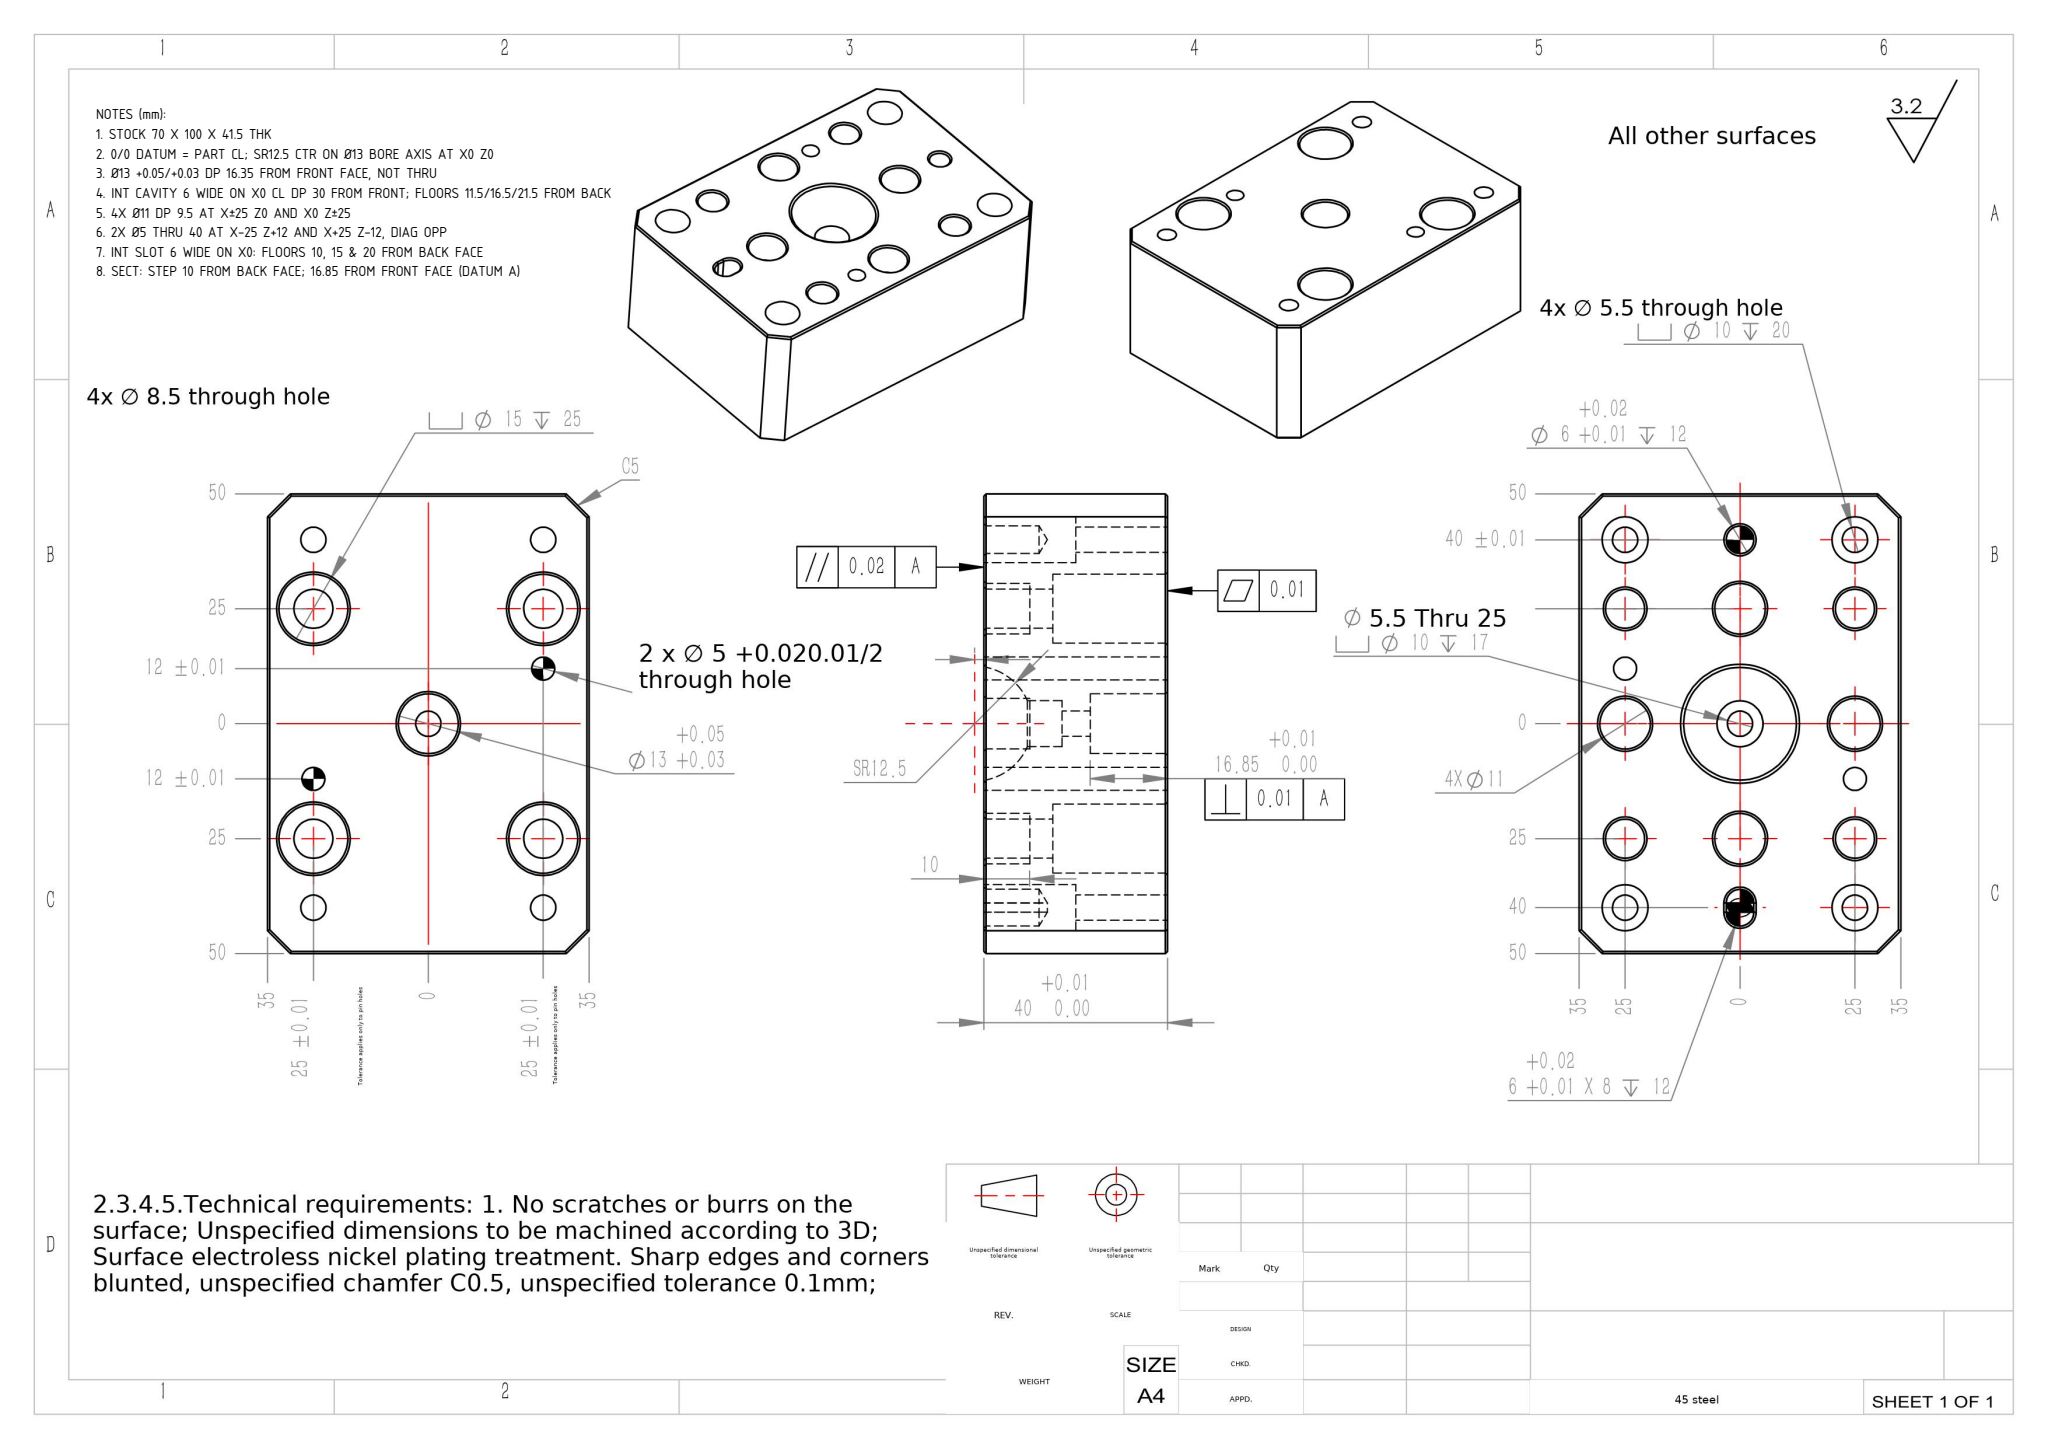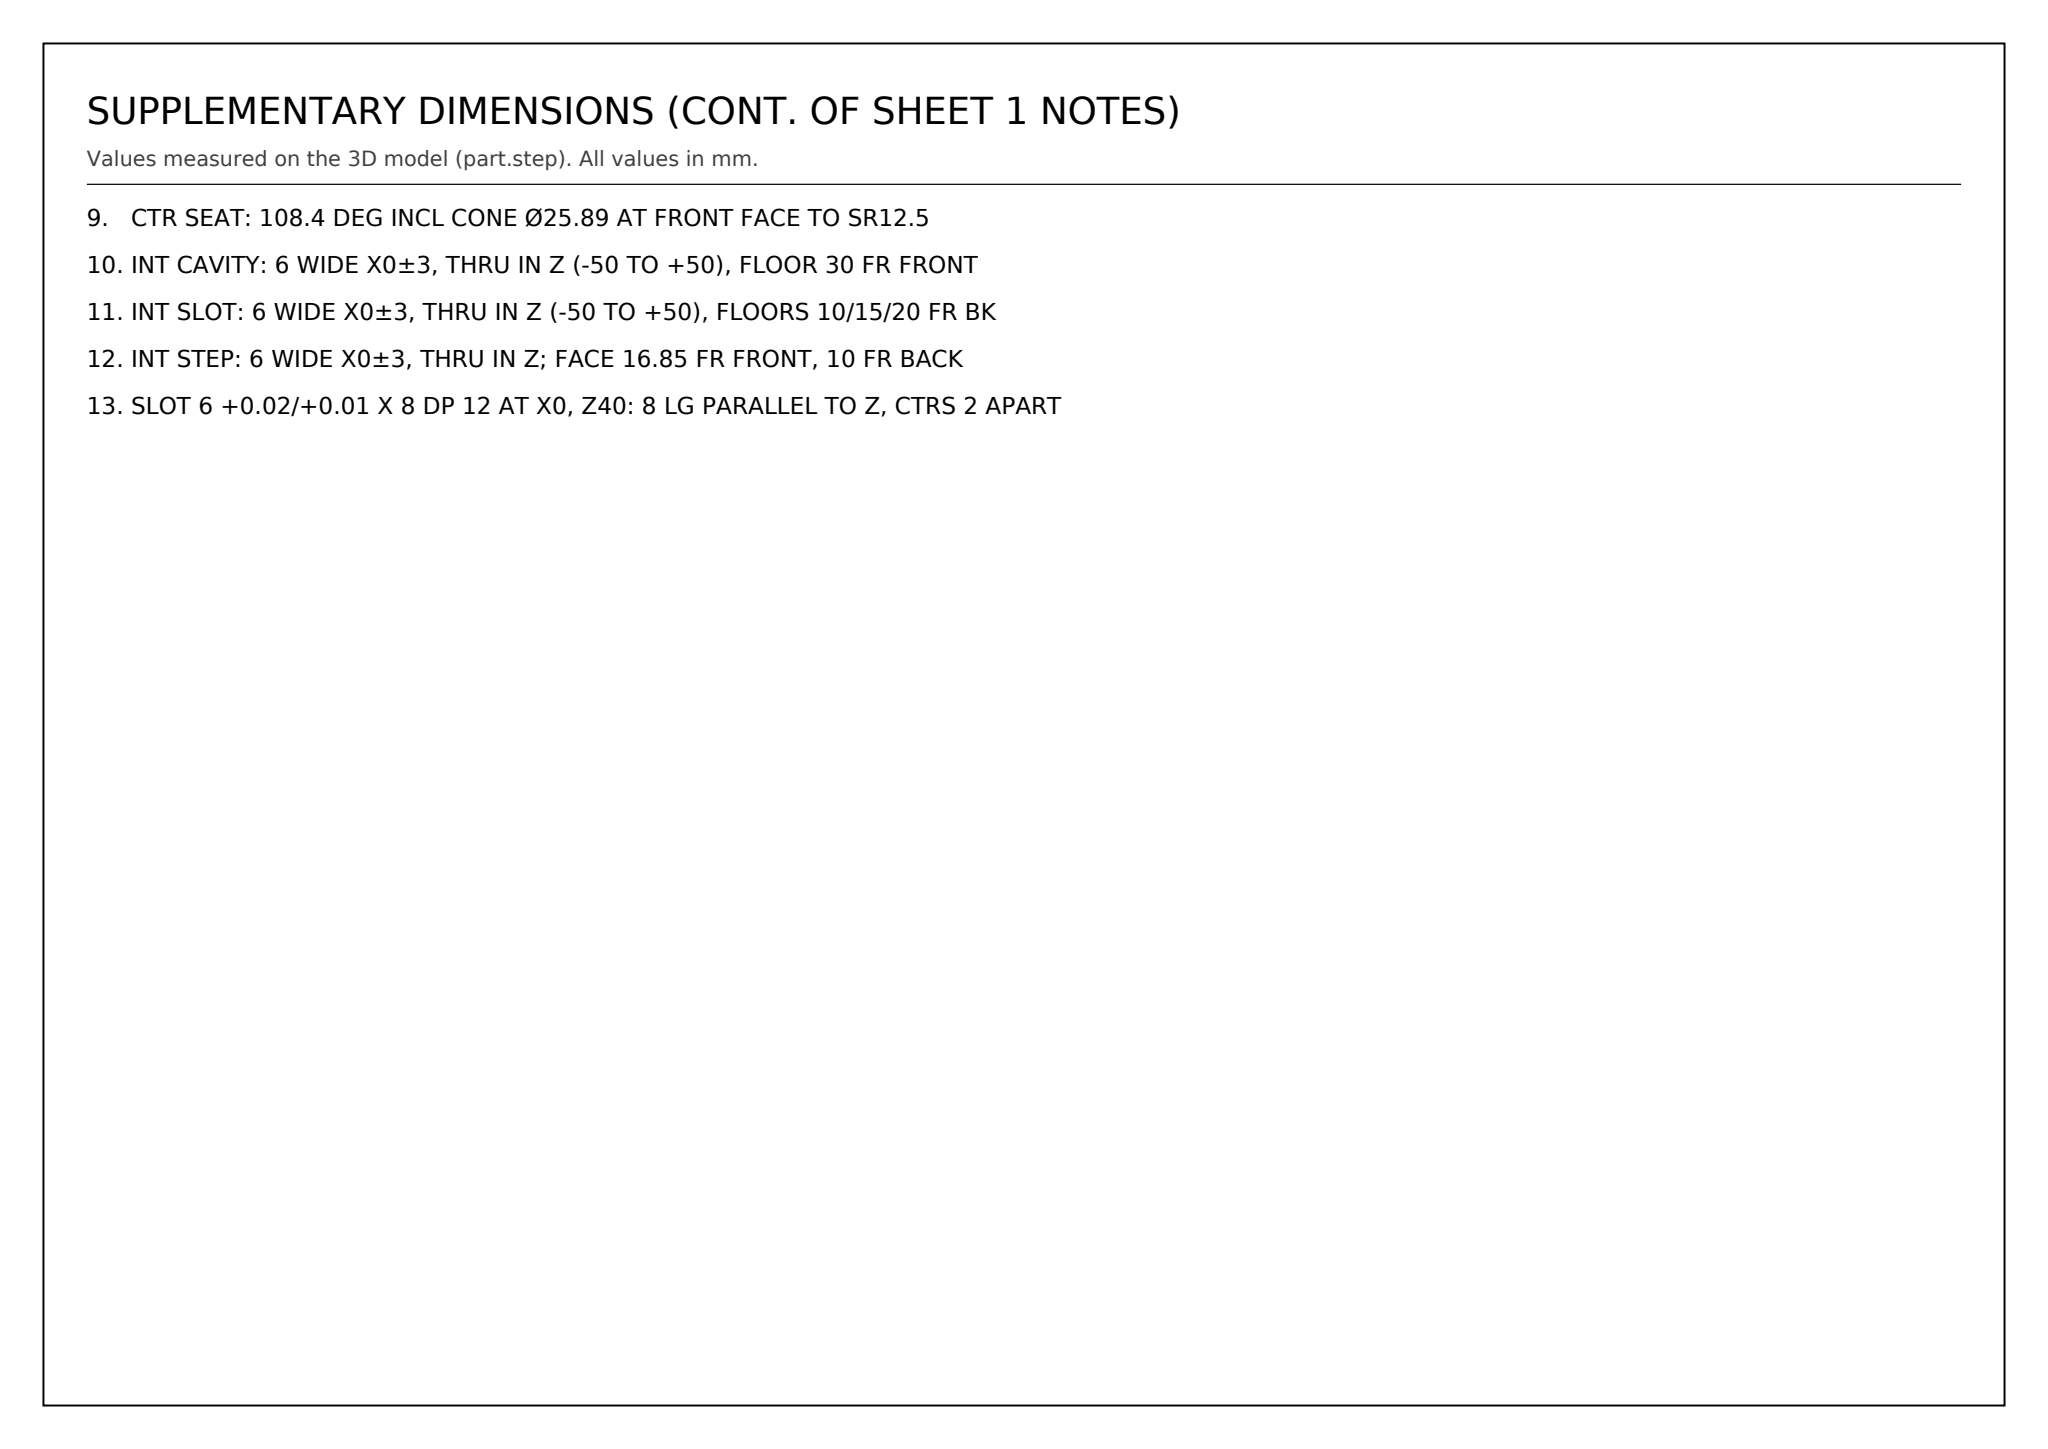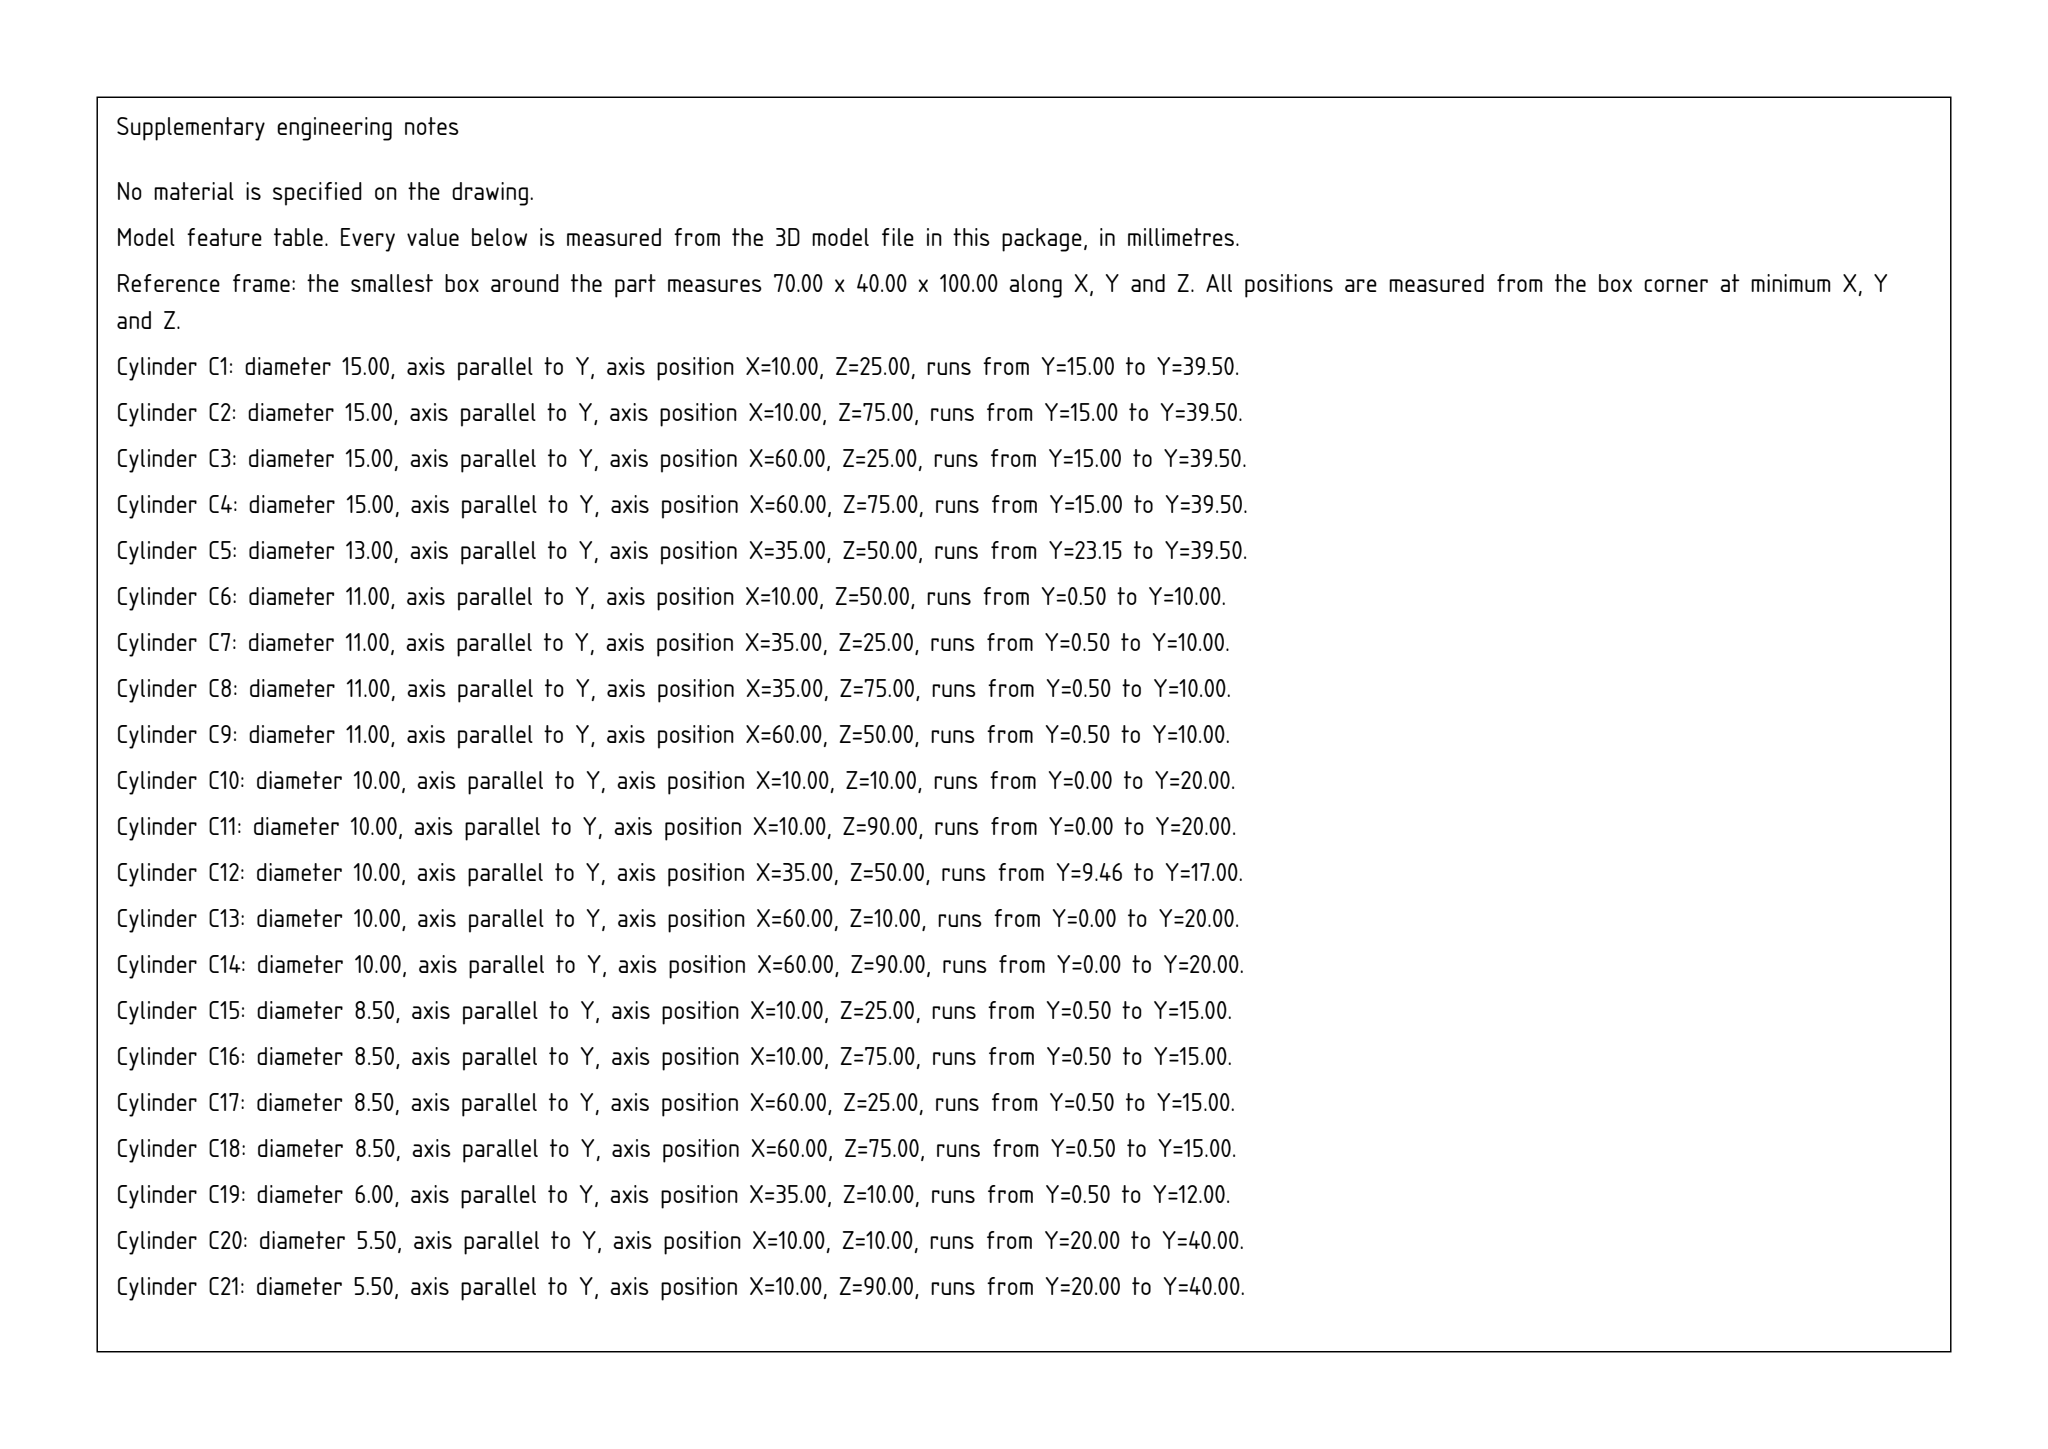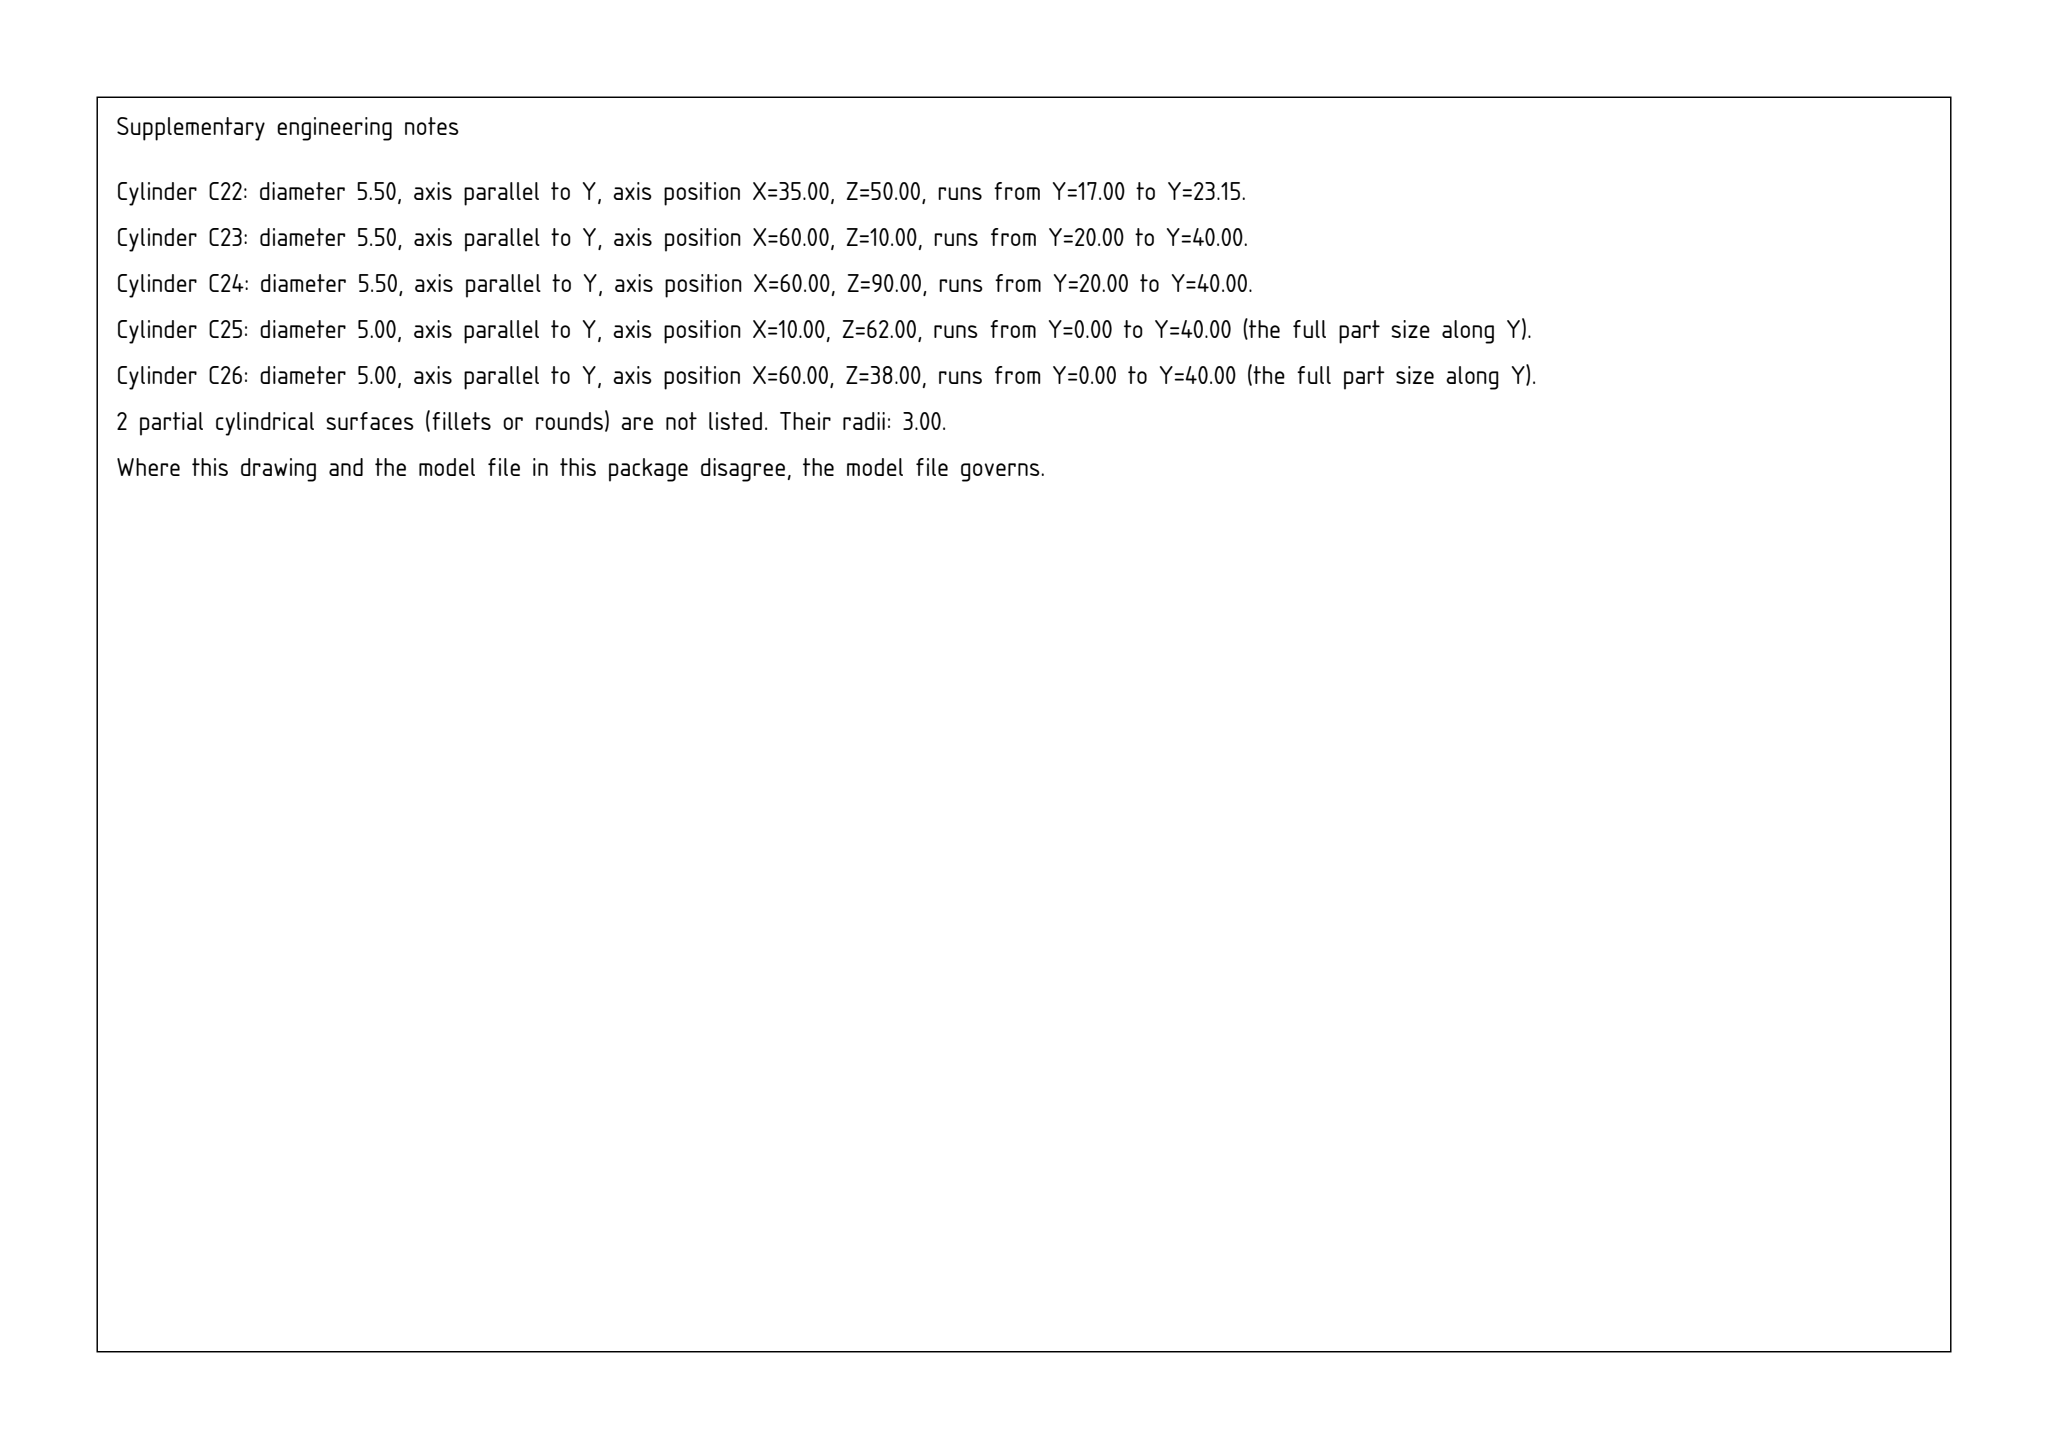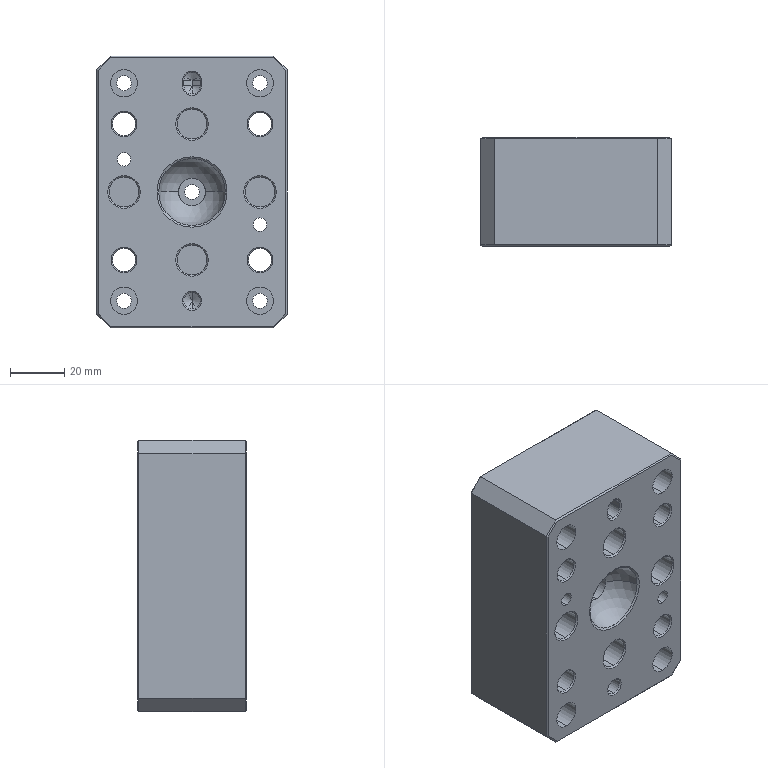Part | SolidWorks | mm | 1 solid | 141 faces | box 70 x 40 x 100 mm | volume 236290 mm3 | cylinder 55 | plane 46 | cone 38 | sphere 2 | commonest cylinder face diameters 10 x10 5.5 x10 11 x8 15 x8 8.5 x8 6 x5 5 x4 13 x2
Drawing notes:
STOCK 70 X 100 X 41.5 THK | from the solid: bbox_xyz [70.0, 41.5, 100.0]
0/0 DATUM = PART CL; SR12.5 CTR ON Ø13 BORE AXIS AT X0 Z0 | from the solid: Ø13 axis at x=35.0, z=50.0 = bbox centre; cone 108.4 deg ref dia 25.887 coaxial
Ø13 +0.05/+0.03 DP 16.35 FROM FRONT FACE, NOT THRU | from the solid: Ø13 cyl, axis y, pos (35,50), length 16.35
INT CAVITY 6 WIDE ON X0 CL DP 30 FROM FRONT; FLOORS 11.5/16.5/21.5 FROM BACK | from the solid: x planes 32.0 & 38.0 (6 wide, sym about x=35); y planes 11.5, 16.5, 21.5; 41.5-11.5=30
4X Ø11 DP 9.5 AT X±25 Z0 AND X0 Z±25 | from the solid: Ø11 cyls len 9.5 at (10,50),(60,50),(35,25),(35,75); datum x=35, z=50
2X Ø5 THRU 40 AT X-25 Z+12 AND X+25 Z-12, DIAG OPP | from the solid: Ø5 cyls len 40 at (10,62) and (60,38); datum x=35, z=50
INT SLOT 6 WIDE ON X0: FLOORS 10, 15 & 20 FROM BACK FACE | from the solid: Slot walls = planes x=32.0 & x=38.0 (6 wide, centred on X35 = X0 CL); three floor planes y=11.5/16.5/21.5 vs back face y=1.5 (front face y=41.5, 40 thk) -> 10/15/20 deep
SECT: STEP 10 FROM BACK FACE; 16.85 FROM FRONT FACE (DATUM A) | from the solid: Plane y=11.5 is 10.0 from back face y=1.5; plane y=24.65 is 16.85 from front face y=41.5 (matches 16.85 +0.01/0)
CTR SEAT: 108.4 DEG INCL CONE Ø25.89 AT FRONT FACE TO SR12.5 | from the solid: cones[108.4, ref_dia 25.887] concentric with central Ø13/Ø10/Ø5.5 bores at x=35, z=50 (X0,Z0); opens on front face y=41.5
INT CAVITY: 6 WIDE X0±3, THRU IN Z (-50 TO +50), FLOOR 30 FR FRONT | from the solid: Planes x=32 & x=38 (one face each) = 6 wide ctr X35 (X0); no internal z-normal planes, only z=0 & z=100 end faces -> channel runs full 100 length; floor y=11.5 = 30 from front face y=41.5
INT SLOT: 6 WIDE X0±3, THRU IN Z (-50 TO +50), FLOORS 10/15/20 FR BK | from the solid: Same 6 wide walls x=32/38; floor planes y=11.5, 16.5, 21.5 = 10/15/20 from back ref face y=1.5; no z-normal internal planes -> thru in Z
INT STEP: 6 WIDE X0±3, THRU IN Z; FACE 16.85 FR FRONT, 10 FR BACK | from the solid: Step faces y=24.65 (41.5-24.65=16.85 from front) and y=11.5 (10 from back ref y=1.5); X limits x=32/38; no z-normal internal planes
SLOT 6 +0.02/+0.01 X 8 DP 12 AT X0, Z40: 8 LG PARALLEL TO Z, CTRS 2 APART | from the solid: Ø6 cyls y-axis at x=35, z=89 and z=91, len 11.5; end ctrs 2 apart in Z, 6+2=8 overall along Z, ctr z=90 = Z40 from CL z=50